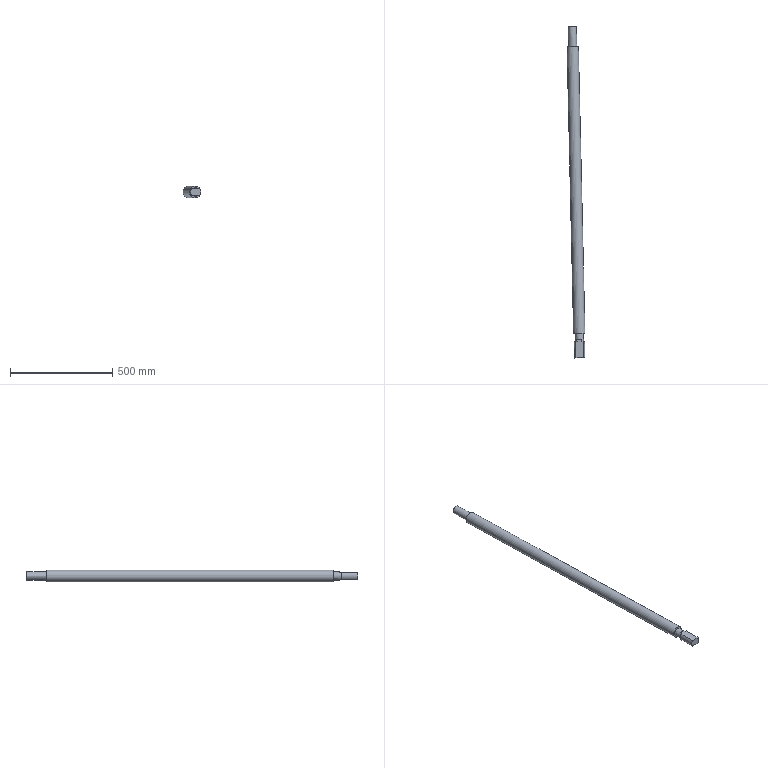Component | NX | 6 | 1 solid | 16 faces | volume 3740922 mm3 | plane 10 | cylinder 5 | cone 1 | commonest cylinder face diameters 40 x2 50 x2 56 x1